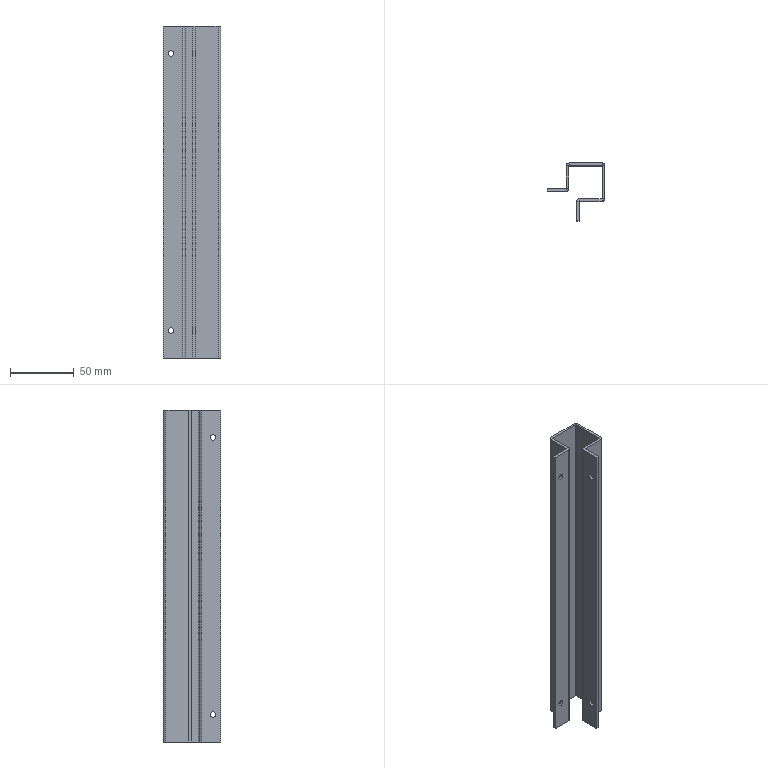Component | SolidWorks | Cover1-2XG1-1 | 1 solid | 54 faces | volume 65277 mm3 | plane 36 | cylinder 18 | commonest cylinder face diameters 4.2 x8 4.1 x5 0.1 x5